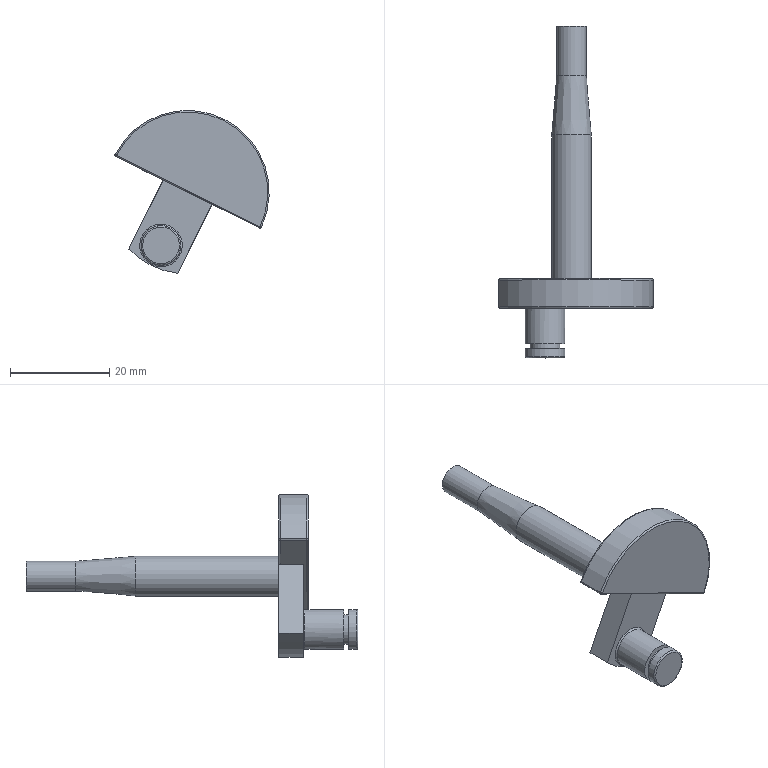Component | NX | CRANKSHAFT | 1 solid | 31 faces | volume 6189 mm3 | cylinder 12 | plane 10 | sphere 4 | torus 4 | cone 1 | commonest cylinder face diameters 0.6 x5 8 x3 6 x2 33 x2